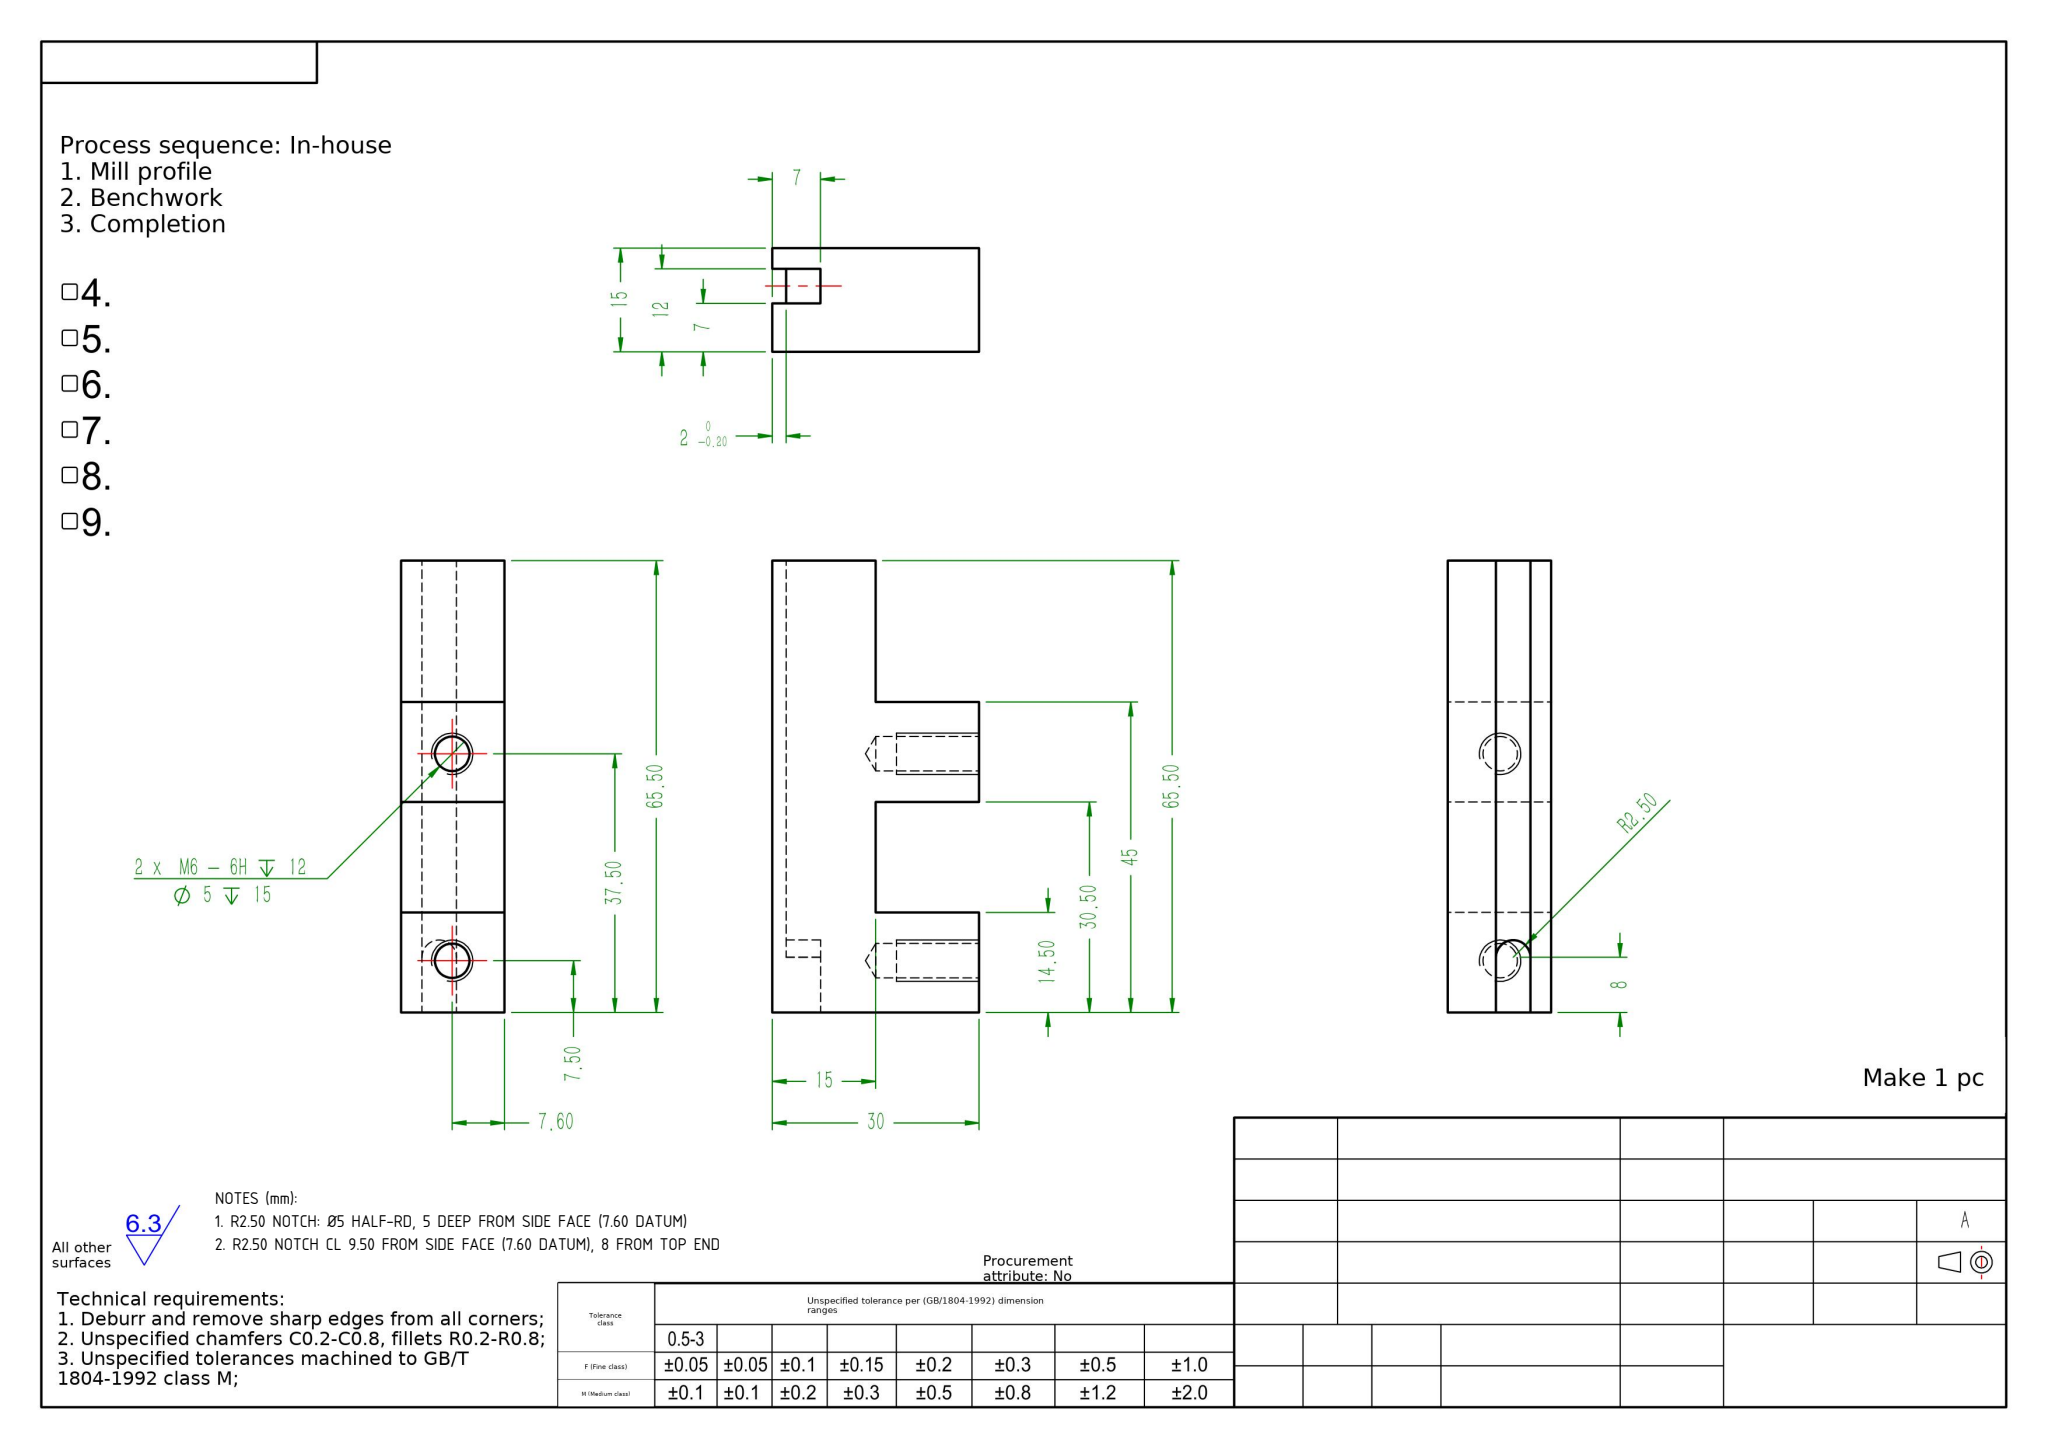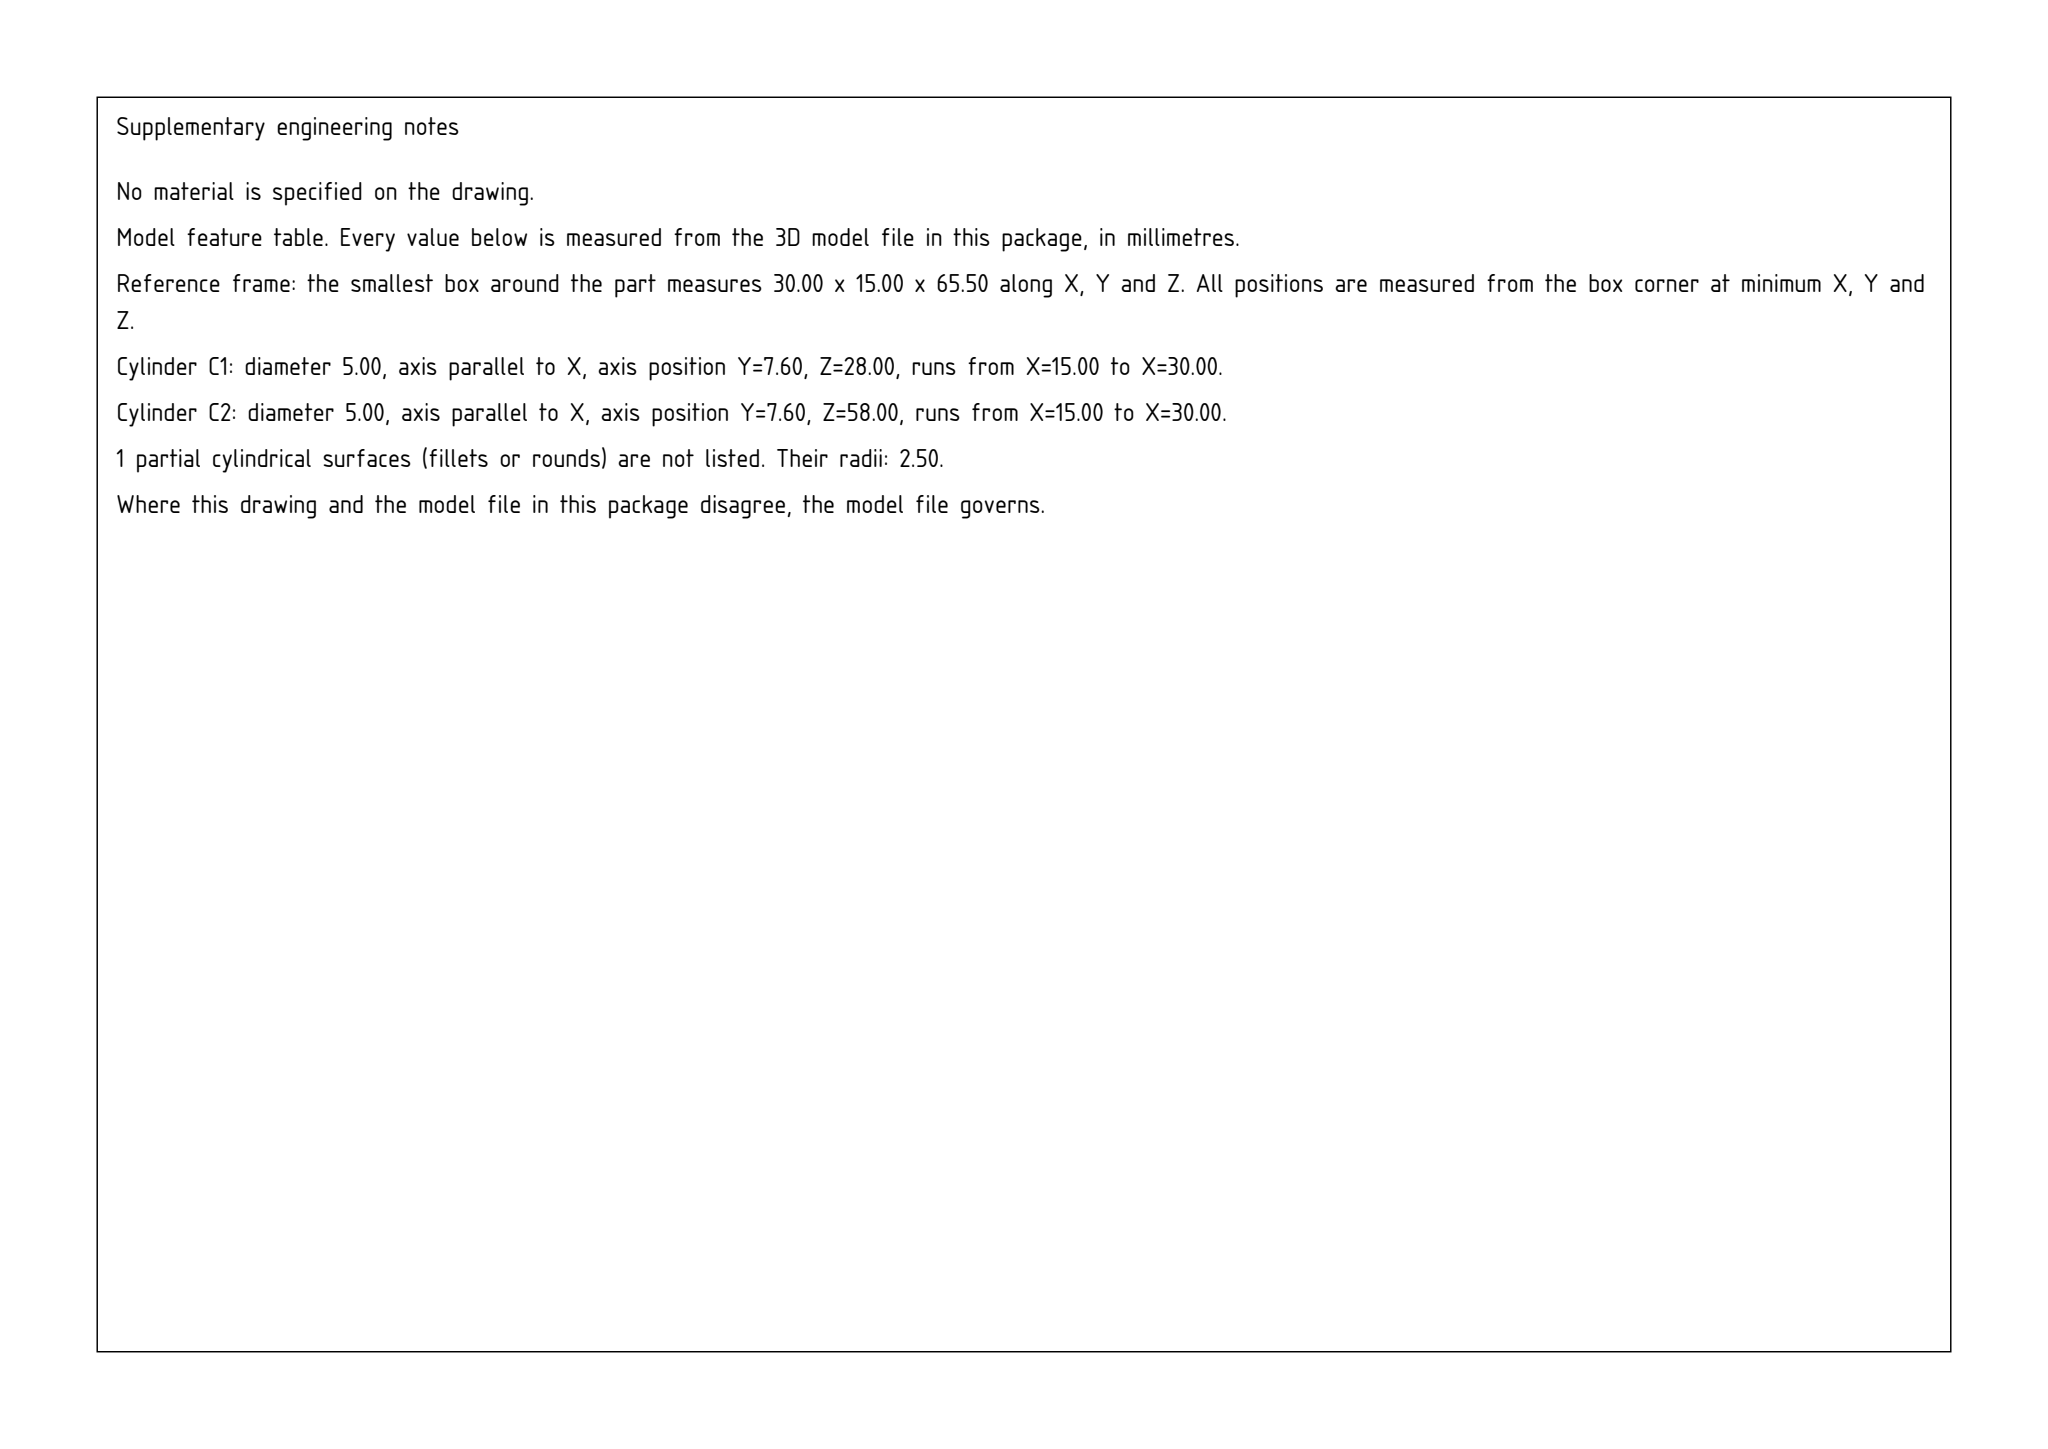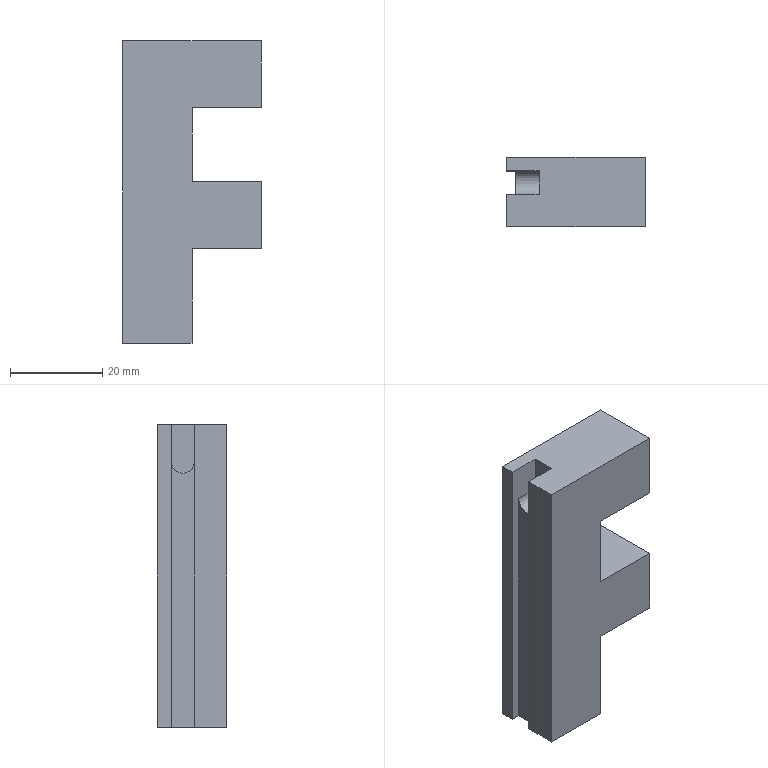Part | SolidWorks | mm | 1 solid | 26 faces | box 30 x 15 x 65.5 mm | volume 19750 mm3 | plane 17 | cylinder 5 | cone 4 | commonest cylinder face diameters 5 x5
Drawing notes:
R2.50 NOTCH: Ø5 HALF-RD, 5 DEEP FROM SIDE FACE (7.60 DATUM) | from the solid: cylinder dia 5.0, axis x, length 5.0 starting at x=0 face
R2.50 NOTCH CL 9.50 FROM SIDE FACE (7.60 DATUM), 8 FROM TOP END | from the solid: cylinder [5.0,'x',[null,9.5,57.5],5.0]; 65.5-57.5=8
build123d program:
from build123d import *

# Parameters (mm, degrees)
BOSS_EXTRUDE1_DEPTH   = 15
M6_TAPPED_HOLE1_D     = 5
M6_TAPPED_HOLE1_DEPTH = 15
M6_TAPPED_HOLE1_TIP   = 1.502
SKETCH4_W             = 65.5
SKETCH4_H             = 5
CUT_EXTRUDE1_DEPTH    = 2
CUT_EXTRUDE2_DEPTH    = 5


with BuildPart() as part:
    # Sketch1 → Boss-Extrude1 (new body)
    with BuildSketch(Plane(origin=(0, 0, 0), x_dir=(1, 0, 0), z_dir=(0, 1, 0))):
        Polygon((0, 0), (0, 65.5), (15, 65.5), (15, 45), (30, 45), (30, 30.5), (15, 30.5), (15, 14.5), (30, 14.5), (30, 0), align=None)
    extrude(amount=BOSS_EXTRUDE1_DEPTH)

    # M6 Tapped Hole1
    with Locations(Plane(origin=(30, 0, 0), x_dir=(0, 0, -1), z_dir=(1, 0, 0))):
        with Locations((7.5, 7.6), (37.5, 7.6)):
            Hole(M6_TAPPED_HOLE1_D / 2, depth=M6_TAPPED_HOLE1_DEPTH)
            with Locations((0, 0, -(M6_TAPPED_HOLE1_DEPTH + M6_TAPPED_HOLE1_TIP / 2))):  # 118° drill point
                Cone(0, M6_TAPPED_HOLE1_D / 2, M6_TAPPED_HOLE1_TIP, mode=Mode.SUBTRACT)

    # Sketch4 → Cut-Extrude1 (cut)
    with BuildSketch(Plane.ZY):
        with Locations((-32.75, 9.5)):
            Rectangle(SKETCH4_W, SKETCH4_H)
    extrude(amount=-CUT_EXTRUDE1_DEPTH, mode=Mode.SUBTRACT)

    # Sketch5 → Cut-Extrude2 (cut)
    with BuildSketch(Plane.ZY.offset(-2)):
        with BuildLine():
            Line((0, 7), (-8, 7))
            ThreePointArc((-8, 7), (-10.5, 9.5), (-8, 12))
            Line((-8, 12), (0, 12))
            ThreePointArc((0, 12), (2.5, 9.5), (0, 7))
        make_face()
    extrude(amount=-CUT_EXTRUDE2_DEPTH, mode=Mode.SUBTRACT)


solid = part.part
STEP:
#1=CARTESIAN_POINT('',(15.,7.6,-5.));
#2=VERTEX_POINT('',#1);
#3=CARTESIAN_POINT('',(15.,7.6,-10.));
#4=VERTEX_POINT('',#3);
#5=CARTESIAN_POINT('',(15.,7.6,-7.5));
#6=DIRECTION('',(1.,0.,-0.));
#7=DIRECTION('',(0.,0.,-1.));
#8=AXIS2_PLACEMENT_3D('',#5,#6,#7);
#9=CIRCLE('',#8,2.5);
#10=EDGE_CURVE('',#2,#4,#9,.T.);
#11=ORIENTED_EDGE('',*,*,#10,.F.);
#12=CARTESIAN_POINT('',(30.,7.6,-5.));
#13=VERTEX_POINT('',#12);
#14=CARTESIAN_POINT('',(30.,7.6,-5.));
#15=DIRECTION('',(1.,0.,-0.));
#16=VECTOR('',#15,1000.);
#17=LINE('',#14,#16);
#18=EDGE_CURVE('',#2,#13,#17,.T.);
#19=ORIENTED_EDGE('',*,*,#18,.T.);
#20=CARTESIAN_POINT('',(30.,7.6,-10.));
#21=VERTEX_POINT('',#20);
#22=CARTESIAN_POINT('',(30.,7.6,-7.5));
#23=DIRECTION('',(1.,0.,-0.));
#24=DIRECTION('',(0.,0.,-1.));
#25=AXIS2_PLACEMENT_3D('',#22,#23,#24);
#26=CIRCLE('',#25,2.5);
#27=EDGE_CURVE('',#13,#21,#26,.T.);
#28=ORIENTED_EDGE('',*,*,#27,.T.);
#29=CARTESIAN_POINT('',(30.,7.6,-10.));
#30=DIRECTION('',(1.,0.,-0.));
#31=VECTOR('',#30,1000.);
#32=LINE('',#29,#31);
#33=EDGE_CURVE('',#4,#21,#32,.T.);
#34=ORIENTED_EDGE('',*,*,#33,.F.);
#35=EDGE_LOOP('',(#11,#19,#28,#34));
#36=FACE_OUTER_BOUND('',#35,.T.);
#37=CARTESIAN_POINT('',(30.,7.6,-7.5));
#38=DIRECTION('',(1.,0.,-0.));
#39=DIRECTION('',(0.,0.,-1.));
#40=AXIS2_PLACEMENT_3D('',#37,#38,#39);
#41=CYLINDRICAL_SURFACE('',#40,2.5);
#42=ADVANCED_FACE('',(#36),#41,.F.);
#43=CARTESIAN_POINT('',(13.498,7.6,-7.5));
#44=VERTEX_POINT('',#43);
#45=CARTESIAN_POINT('',(15.,7.6,-10.));
#46=DIRECTION('',(0.515,0.,-0.8572));
#47=VECTOR('',#46,1000.);
#48=LINE('',#45,#47);
#49=EDGE_CURVE('',#44,#4,#48,.T.);
#50=ORIENTED_EDGE('',*,*,#49,.F.);
#51=CARTESIAN_POINT('',(15.,7.6,-5.));
#52=DIRECTION('',(0.515,0.,0.8572));
#53=VECTOR('',#52,1000.);
#54=LINE('',#51,#53);
#55=EDGE_CURVE('',#44,#2,#54,.T.);
#56=ORIENTED_EDGE('',*,*,#55,.T.);
#57=ORIENTED_EDGE('',*,*,#10,.T.);
#58=EDGE_LOOP('',(#50,#56,#57));
#59=FACE_OUTER_BOUND('',#58,.T.);
#60=CARTESIAN_POINT('',(15.,7.6,-7.5));
#61=DIRECTION('',(1.,0.,-0.));
#62=DIRECTION('',(0.,0.,-1.));
#63=AXIS2_PLACEMENT_3D('',#60,#61,#62);
#64=CONICAL_SURFACE('',#63,2.5,1.03);
#65=ADVANCED_FACE('',(#59),#64,.F.);
#66=CARTESIAN_POINT('',(15.,7.6,-35.));
#67=VERTEX_POINT('',#66);
#68=CARTESIAN_POINT('',(15.,7.6,-40.));
#69=VERTEX_POINT('',#68);
#70=CARTESIAN_POINT('',(15.,7.6,-37.5));
#71=DIRECTION('',(1.,0.,-0.));
#72=DIRECTION('',(0.,0.,-1.));
#73=AXIS2_PLACEMENT_3D('',#70,#71,#72);
#74=CIRCLE('',#73,2.5);
#75=EDGE_CURVE('',#67,#69,#74,.T.);
#76=ORIENTED_EDGE('',*,*,#75,.F.);
#77=CARTESIAN_POINT('',(30.,7.6,-35.));
#78=VERTEX_POINT('',#77);
#79=CARTESIAN_POINT('',(30.,7.6,-35.));
#80=DIRECTION('',(1.,0.,-0.));
#81=VECTOR('',#80,1000.);
#82=LINE('',#79,#81);
#83=EDGE_CURVE('',#67,#78,#82,.T.);
#84=ORIENTED_EDGE('',*,*,#83,.T.);
#85=CARTESIAN_POINT('',(30.,7.6,-40.));
#86=VERTEX_POINT('',#85);
#87=CARTESIAN_POINT('',(30.,7.6,-37.5));
#88=DIRECTION('',(1.,0.,-0.));
#89=DIRECTION('',(0.,0.,-1.));
#90=AXIS2_PLACEMENT_3D('',#87,#88,#89);
#91=CIRCLE('',#90,2.5);
#92=EDGE_CURVE('',#78,#86,#91,.T.);
#93=ORIENTED_EDGE('',*,*,#92,.T.);
#94=CARTESIAN_POINT('',(30.,7.6,-40.));
#95=DIRECTION('',(1.,0.,-0.));
#96=VECTOR('',#95,1000.);
#97=LINE('',#94,#96);
#98=EDGE_CURVE('',#69,#86,#97,.T.);
#99=ORIENTED_EDGE('',*,*,#98,.F.);
#100=EDGE_LOOP('',(#76,#84,#93,#99));
#101=FACE_OUTER_BOUND('',#100,.T.);
#102=CARTESIAN_POINT('',(30.,7.6,-37.5));
#103=DIRECTION('',(1.,0.,-0.));
#104=DIRECTION('',(0.,0.,-1.));
#105=AXIS2_PLACEMENT_3D('',#102,#103,#104);
#106=CYLINDRICAL_SURFACE('',#105,2.5);
#107=ADVANCED_FACE('',(#101),#106,.F.);
#108=CARTESIAN_POINT('',(13.498,7.6,-37.5));
#109=VERTEX_POINT('',#108);
#110=CARTESIAN_POINT('',(15.,7.6,-40.));
#111=DIRECTION('',(0.515,0.,-0.8572));
#112=VECTOR('',#111,1000.);
#113=LINE('',#110,#112);
#114=EDGE_CURVE('',#109,#69,#113,.T.);
#115=ORIENTED_EDGE('',*,*,#114,.F.);
#116=CARTESIAN_POINT('',(15.,7.6,-35.));
#117=DIRECTION('',(0.515,0.,0.8572));
#118=VECTOR('',#117,1000.);
#119=LINE('',#116,#118);
#120=EDGE_CURVE('',#109,#67,#119,.T.);
#121=ORIENTED_EDGE('',*,*,#120,.T.);
#122=ORIENTED_EDGE('',*,*,#75,.T.);
#123=EDGE_LOOP('',(#115,#121,#122));
#124=FACE_OUTER_BOUND('',#123,.T.);
#125=CARTESIAN_POINT('',(15.,7.6,-37.5));
#126=DIRECTION('',(1.,0.,-0.));
#127=DIRECTION('',(0.,0.,-1.));
#128=AXIS2_PLACEMENT_3D('',#125,#126,#127);
#129=CONICAL_SURFACE('',#128,2.5,1.03);
#130=ADVANCED_FACE('',(#124),#129,.F.);
#131=CARTESIAN_POINT('',(0.,15.,-65.5));
#132=VERTEX_POINT('',#131);
#133=CARTESIAN_POINT('',(0.,12.,-65.5));
#134=VERTEX_POINT('',#133);
#135=CARTESIAN_POINT('',(0.,15.,-65.5));
#136=DIRECTION('',(0.,-1.,0.));
#137=VECTOR('',#136,1000.);
#138=LINE('',#135,#137);
#139=EDGE_CURVE('',#132,#134,#138,.T.);
#140=ORIENTED_EDGE('',*,*,#139,.T.);
#141=CARTESIAN_POINT('',(0.,12.,0.));
#142=VERTEX_POINT('',#141);
#143=CARTESIAN_POINT('',(0.,12.,-65.5));
#144=DIRECTION('',(0.,0.,-1.));
#145=VECTOR('',#144,1000.);
#146=LINE('',#143,#145);
#147=EDGE_CURVE('',#142,#134,#146,.T.);
#148=ORIENTED_EDGE('',*,*,#147,.F.);
#149=CARTESIAN_POINT('',(0.,15.,0.));
#150=VERTEX_POINT('',#149);
#151=CARTESIAN_POINT('',(0.,15.,0.));
#152=DIRECTION('',(0.,-1.,0.));
#153=VECTOR('',#152,1000.);
#154=LINE('',#151,#153);
#155=EDGE_CURVE('',#150,#142,#154,.T.);
#156=ORIENTED_EDGE('',*,*,#155,.F.);
#157=CARTESIAN_POINT('',(0.,15.,0.));
#158=DIRECTION('',(0.,0.,1.));
#159=VECTOR('',#158,1000.);
#160=LINE('',#157,#159);
#161=EDGE_CURVE('',#132,#150,#160,.T.);
#162=ORIENTED_EDGE('',*,*,#161,.F.);
#163=EDGE_LOOP('',(#140,#148,#156,#162));
#164=FACE_OUTER_BOUND('',#163,.T.);
#165=CARTESIAN_POINT('',(0.,15.,0.));
#166=DIRECTION('',(1.,0.,0.));
#167=DIRECTION('',(0.,0.,-1.));
#168=AXIS2_PLACEMENT_3D('',#165,#166,#167);
#169=PLANE('',#168);
#170=ADVANCED_FACE('',(#164),#169,.F.);
#171=CARTESIAN_POINT('',(7.,7.,0.));
#172=VERTEX_POINT('',#171);
#173=CARTESIAN_POINT('',(7.,12.,0.));
#174=VERTEX_POINT('',#173);
#175=CARTESIAN_POINT('',(7.,15.,0.));
#176=DIRECTION('',(0.,1.,0.));
#177=VECTOR('',#176,1000.);
#178=LINE('',#175,#177);
#179=EDGE_CURVE('',#172,#174,#178,.T.);
#180=ORIENTED_EDGE('',*,*,#179,.F.);
#181=CARTESIAN_POINT('',(0.,7.,0.));
#182=VERTEX_POINT('',#181);
#183=CARTESIAN_POINT('',(2.,7.,0.));
#184=DIRECTION('',(-1.,0.,0.));
#185=VECTOR('',#184,1000.);
#186=LINE('',#183,#185);
#187=EDGE_CURVE('',#172,#182,#186,.T.);
#188=ORIENTED_EDGE('',*,*,#187,.T.);
#189=CARTESIAN_POINT('',(0.,0.,0.));
#190=VERTEX_POINT('',#189);
#191=CARTESIAN_POINT('',(0.,15.,0.));
#192=DIRECTION('',(0.,-1.,0.));
#193=VECTOR('',#192,1000.);
#194=LINE('',#191,#193);
#195=EDGE_CURVE('',#182,#190,#194,.T.);
#196=ORIENTED_EDGE('',*,*,#195,.T.);
#197=CARTESIAN_POINT('',(30.,0.,0.));
#198=VERTEX_POINT('',#197);
#199=CARTESIAN_POINT('',(30.,0.,0.));
#200=DIRECTION('',(1.,0.,0.));
#201=VECTOR('',#200,1000.);
#202=LINE('',#199,#201);
#203=EDGE_CURVE('',#190,#198,#202,.T.);
#204=ORIENTED_EDGE('',*,*,#203,.T.);
#205=CARTESIAN_POINT('',(30.,15.,0.));
#206=VERTEX_POINT('',#205);
#207=CARTESIAN_POINT('',(30.,15.,0.));
#208=DIRECTION('',(0.,-1.,0.));
#209=VECTOR('',#208,1000.);
#210=LINE('',#207,#209);
#211=EDGE_CURVE('',#206,#198,#210,.T.);
#212=ORIENTED_EDGE('',*,*,#211,.F.);
#213=CARTESIAN_POINT('',(30.,15.,0.));
#214=DIRECTION('',(1.,0.,0.));
#215=VECTOR('',#214,1000.);
#216=LINE('',#213,#215);
#217=EDGE_CURVE('',#150,#206,#216,.T.);
#218=ORIENTED_EDGE('',*,*,#217,.F.);
#219=ORIENTED_EDGE('',*,*,#155,.T.);
#220=CARTESIAN_POINT('',(2.,12.,0.));
#221=DIRECTION('',(-1.,0.,0.));
#222=VECTOR('',#221,1000.);
#223=LINE('',#220,#222);
#224=EDGE_CURVE('',#174,#142,#223,.T.);
#225=ORIENTED_EDGE('',*,*,#224,.F.);
#226=EDGE_LOOP('',(#180,#188,#196,#204,#212,#218,#219,#225));
#227=FACE_OUTER_BOUND('',#226,.T.);
#228=CARTESIAN_POINT('',(30.,15.,0.));
#229=DIRECTION('',(0.,0.,-1.));
#230=DIRECTION('',(-1.,0.,-0.));
#231=AXIS2_PLACEMENT_3D('',#228,#229,#230);
#232=PLANE('',#231);
#233=ADVANCED_FACE('',(#227),#232,.F.);
#234=CARTESIAN_POINT('',(30.,7.6,-7.5));
#235=DIRECTION('',(1.,0.,-0.));
#236=DIRECTION('',(0.,0.,-1.));
#237=AXIS2_PLACEMENT_3D('',#234,#235,#236);
#238=CIRCLE('',#237,2.5);
#239=EDGE_CURVE('',#21,#13,#238,.T.);
#240=ORIENTED_EDGE('',*,*,#239,.F.);
#241=ORIENTED_EDGE('',*,*,#27,.F.);
#242=EDGE_LOOP('',(#240,#241));
#243=FACE_BOUND('',#242,.T.);
#244=CARTESIAN_POINT('',(30.,0.,-14.5));
#245=VERTEX_POINT('',#244);
#246=CARTESIAN_POINT('',(30.,0.,-14.5));
#247=DIRECTION('',(-0.,0.,-1.));
#248=VECTOR('',#247,1000.);
#249=LINE('',#246,#248);
#250=EDGE_CURVE('',#198,#245,#249,.T.);
#251=ORIENTED_EDGE('',*,*,#250,.T.);
#252=CARTESIAN_POINT('',(30.,15.,-14.5));
#253=VERTEX_POINT('',#252);
#254=CARTESIAN_POINT('',(30.,15.,-14.5));
#255=DIRECTION('',(0.,-1.,0.));
#256=VECTOR('',#255,1000.);
#257=LINE('',#254,#256);
#258=EDGE_CURVE('',#253,#245,#257,.T.);
#259=ORIENTED_EDGE('',*,*,#258,.F.);
#260=CARTESIAN_POINT('',(30.,15.,-14.5));
#261=DIRECTION('',(-0.,0.,-1.));
#262=VECTOR('',#261,1000.);
#263=LINE('',#260,#262);
#264=EDGE_CURVE('',#206,#253,#263,.T.);
#265=ORIENTED_EDGE('',*,*,#264,.F.);
#266=ORIENTED_EDGE('',*,*,#211,.T.);
#267=EDGE_LOOP('',(#251,#259,#265,#266));
#268=FACE_OUTER_BOUND('',#267,.T.);
#269=CARTESIAN_POINT('',(30.,15.,-14.5));
#270=DIRECTION('',(-1.,0.,0.));
#271=DIRECTION('',(0.,0.,1.));
#272=AXIS2_PLACEMENT_3D('',#269,#270,#271);
#273=PLANE('',#272);
#274=ADVANCED_FACE('',(#243,#268),#273,.F.);
#275=CARTESIAN_POINT('',(15.,0.,-14.5));
#276=VERTEX_POINT('',#275);
#277=CARTESIAN_POINT('',(15.,0.,-14.5));
#278=DIRECTION('',(-1.,0.,0.));
#279=VECTOR('',#278,1000.);
#280=LINE('',#277,#279);
#281=EDGE_CURVE('',#245,#276,#280,.T.);
#282=ORIENTED_EDGE('',*,*,#281,.T.);
#283=CARTESIAN_POINT('',(15.,15.,-14.5));
#284=VERTEX_POINT('',#283);
#285=CARTESIAN_POINT('',(15.,15.,-14.5));
#286=DIRECTION('',(0.,-1.,0.));
#287=VECTOR('',#286,1000.);
#288=LINE('',#285,#287);
#289=EDGE_CURVE('',#284,#276,#288,.T.);
#290=ORIENTED_EDGE('',*,*,#289,.F.);
#291=CARTESIAN_POINT('',(15.,15.,-14.5));
#292=DIRECTION('',(-1.,0.,0.));
#293=VECTOR('',#292,1000.);
#294=LINE('',#291,#293);
#295=EDGE_CURVE('',#253,#284,#294,.T.);
#296=ORIENTED_EDGE('',*,*,#295,.F.);
#297=ORIENTED_EDGE('',*,*,#258,.T.);
#298=EDGE_LOOP('',(#282,#290,#296,#297));
#299=FACE_OUTER_BOUND('',#298,.T.);
#300=CARTESIAN_POINT('',(15.,15.,-14.5));
#301=DIRECTION('',(0.,0.,1.));
#302=DIRECTION('',(1.,0.,0.));
#303=AXIS2_PLACEMENT_3D('',#300,#301,#302);
#304=PLANE('',#303);
#305=ADVANCED_FACE('',(#299),#304,.F.);
#306=CARTESIAN_POINT('',(15.,0.,-30.5));
#307=VERTEX_POINT('',#306);
#308=CARTESIAN_POINT('',(15.,0.,-30.5));
#309=DIRECTION('',(-0.,0.,-1.));
#310=VECTOR('',#309,1000.);
#311=LINE('',#308,#310);
#312=EDGE_CURVE('',#276,#307,#311,.T.);
#313=ORIENTED_EDGE('',*,*,#312,.T.);
#314=CARTESIAN_POINT('',(15.,15.,-30.5));
#315=VERTEX_POINT('',#314);
#316=CARTESIAN_POINT('',(15.,15.,-30.5));
#317=DIRECTION('',(0.,-1.,0.));
#318=VECTOR('',#317,1000.);
#319=LINE('',#316,#318);
#320=EDGE_CURVE('',#315,#307,#319,.T.);
#321=ORIENTED_EDGE('',*,*,#320,.F.);
#322=CARTESIAN_POINT('',(15.,15.,-30.5));
#323=DIRECTION('',(-0.,0.,-1.));
#324=VECTOR('',#323,1000.);
#325=LINE('',#322,#324);
#326=EDGE_CURVE('',#284,#315,#325,.T.);
#327=ORIENTED_EDGE('',*,*,#326,.F.);
#328=ORIENTED_EDGE('',*,*,#289,.T.);
#329=EDGE_LOOP('',(#313,#321,#327,#328));
#330=FACE_OUTER_BOUND('',#329,.T.);
#331=CARTESIAN_POINT('',(15.,15.,-30.5));
#332=DIRECTION('',(-1.,0.,0.));
#333=DIRECTION('',(0.,0.,1.));
#334=AXIS2_PLACEMENT_3D('',#331,#332,#333);
#335=PLANE('',#334);
#336=ADVANCED_FACE('',(#330),#335,.F.);
#337=CARTESIAN_POINT('',(30.,0.,-30.5));
#338=VERTEX_POINT('',#337);
#339=CARTESIAN_POINT('',(30.,0.,-30.5));
#340=DIRECTION('',(1.,0.,-0.));
#341=VECTOR('',#340,1000.);
#342=LINE('',#339,#341);
#343=EDGE_CURVE('',#307,#338,#342,.T.);
#344=ORIENTED_EDGE('',*,*,#343,.T.);
#345=CARTESIAN_POINT('',(30.,15.,-30.5));
#346=VERTEX_POINT('',#345);
#347=CARTESIAN_POINT('',(30.,15.,-30.5));
#348=DIRECTION('',(0.,-1.,0.));
#349=VECTOR('',#348,1000.);
#350=LINE('',#347,#349);
#351=EDGE_CURVE('',#346,#338,#350,.T.);
#352=ORIENTED_EDGE('',*,*,#351,.F.);
#353=CARTESIAN_POINT('',(30.,15.,-30.5));
#354=DIRECTION('',(1.,0.,-0.));
#355=VECTOR('',#354,1000.);
#356=LINE('',#353,#355);
#357=EDGE_CURVE('',#315,#346,#356,.T.);
#358=ORIENTED_EDGE('',*,*,#357,.F.);
#359=ORIENTED_EDGE('',*,*,#320,.T.);
#360=EDGE_LOOP('',(#344,#352,#358,#359));
#361=FACE_OUTER_BOUND('',#360,.T.);
#362=CARTESIAN_POINT('',(30.,15.,-30.5));
#363=DIRECTION('',(-0.,0.,-1.));
#364=DIRECTION('',(-1.,0.,0.));
#365=AXIS2_PLACEMENT_3D('',#362,#363,#364);
#366=PLANE('',#365);
#367=ADVANCED_FACE('',(#361),#366,.F.);
#368=CARTESIAN_POINT('',(30.,7.6,-37.5));
#369=DIRECTION('',(1.,0.,-0.));
#370=DIRECTION('',(0.,0.,-1.));
#371=AXIS2_PLACEMENT_3D('',#368,#369,#370);
#372=CIRCLE('',#371,2.5);
#373=EDGE_CURVE('',#86,#78,#372,.T.);
#374=ORIENTED_EDGE('',*,*,#373,.F.);
#375=ORIENTED_EDGE('',*,*,#92,.F.);
#376=EDGE_LOOP('',(#374,#375));
#377=FACE_BOUND('',#376,.T.);
#378=CARTESIAN_POINT('',(30.,0.,-45.));
#379=VERTEX_POINT('',#378);
#380=CARTESIAN_POINT('',(30.,0.,-45.));
#381=DIRECTION('',(-0.,0.,-1.));
#382=VECTOR('',#381,1000.);
#383=LINE('',#380,#382);
#384=EDGE_CURVE('',#338,#379,#383,.T.);
#385=ORIENTED_EDGE('',*,*,#384,.T.);
#386=CARTESIAN_POINT('',(30.,15.,-45.));
#387=VERTEX_POINT('',#386);
#388=CARTESIAN_POINT('',(30.,15.,-45.));
#389=DIRECTION('',(0.,-1.,0.));
#390=VECTOR('',#389,1000.);
#391=LINE('',#388,#390);
#392=EDGE_CURVE('',#387,#379,#391,.T.);
#393=ORIENTED_EDGE('',*,*,#392,.F.);
#394=CARTESIAN_POINT('',(30.,15.,-45.));
#395=DIRECTION('',(-0.,0.,-1.));
#396=VECTOR('',#395,1000.);
#397=LINE('',#394,#396);
#398=EDGE_CURVE('',#346,#387,#397,.T.);
#399=ORIENTED_EDGE('',*,*,#398,.F.);
#400=ORIENTED_EDGE('',*,*,#351,.T.);
#401=EDGE_LOOP('',(#385,#393,#399,#400));
#402=FACE_OUTER_BOUND('',#401,.T.);
#403=CARTESIAN_POINT('',(30.,15.,-45.));
#404=DIRECTION('',(-1.,0.,0.));
#405=DIRECTION('',(0.,0.,1.));
#406=AXIS2_PLACEMENT_3D('',#403,#404,#405);
#407=PLANE('',#406);
#408=ADVANCED_FACE('',(#377,#402),#407,.F.);
#409=CARTESIAN_POINT('',(15.,0.,-45.));
#410=VERTEX_POINT('',#409);
#411=CARTESIAN_POINT('',(15.,0.,-45.));
#412=DIRECTION('',(-1.,0.,0.));
#413=VECTOR('',#412,1000.);
#414=LINE('',#411,#413);
#415=EDGE_CURVE('',#379,#410,#414,.T.);
#416=ORIENTED_EDGE('',*,*,#415,.T.);
#417=CARTESIAN_POINT('',(15.,15.,-45.));
#418=VERTEX_POINT('',#417);
#419=CARTESIAN_POINT('',(15.,15.,-45.));
#420=DIRECTION('',(0.,-1.,0.));
#421=VECTOR('',#420,1000.);
#422=LINE('',#419,#421);
#423=EDGE_CURVE('',#418,#410,#422,.T.);
#424=ORIENTED_EDGE('',*,*,#423,.F.);
#425=CARTESIAN_POINT('',(15.,15.,-45.));
#426=DIRECTION('',(-1.,0.,0.));
#427=VECTOR('',#426,1000.);
#428=LINE('',#425,#427);
#429=EDGE_CURVE('',#387,#418,#428,.T.);
#430=ORIENTED_EDGE('',*,*,#429,.F.);
#431=ORIENTED_EDGE('',*,*,#392,.T.);
#432=EDGE_LOOP('',(#416,#424,#430,#431));
#433=FACE_OUTER_BOUND('',#432,.T.);
#434=CARTESIAN_POINT('',(15.,15.,-45.));
#435=DIRECTION('',(0.,0.,1.));
#436=DIRECTION('',(1.,0.,0.));
#437=AXIS2_PLACEMENT_3D('',#434,#435,#436);
#438=PLANE('',#437);
#439=ADVANCED_FACE('',(#433),#438,.F.);
#440=CARTESIAN_POINT('',(15.,0.,-65.5));
#441=VERTEX_POINT('',#440);
#442=CARTESIAN_POINT('',(15.,0.,-65.5));
#443=DIRECTION('',(-0.,0.,-1.));
#444=VECTOR('',#443,1000.);
#445=LINE('',#442,#444);
#446=EDGE_CURVE('',#410,#441,#445,.T.);
#447=ORIENTED_EDGE('',*,*,#446,.T.);
#448=CARTESIAN_POINT('',(15.,15.,-65.5));
#449=VERTEX_POINT('',#448);
#450=CARTESIAN_POINT('',(15.,15.,-65.5));
#451=DIRECTION('',(0.,-1.,0.));
#452=VECTOR('',#451,1000.);
#453=LINE('',#450,#452);
#454=EDGE_CURVE('',#449,#441,#453,.T.);
#455=ORIENTED_EDGE('',*,*,#454,.F.);
#456=CARTESIAN_POINT('',(15.,15.,-65.5));
#457=DIRECTION('',(-0.,0.,-1.));
#458=VECTOR('',#457,1000.);
#459=LINE('',#456,#458);
#460=EDGE_CURVE('',#418,#449,#459,.T.);
#461=ORIENTED_EDGE('',*,*,#460,.F.);
#462=ORIENTED_EDGE('',*,*,#423,.T.);
#463=EDGE_LOOP('',(#447,#455,#461,#462));
#464=FACE_OUTER_BOUND('',#463,.T.);
#465=CARTESIAN_POINT('',(15.,15.,-65.5));
#466=DIRECTION('',(-1.,0.,0.));
#467=DIRECTION('',(0.,0.,1.));
#468=AXIS2_PLACEMENT_3D('',#465,#466,#467);
#469=PLANE('',#468);
#470=ADVANCED_FACE('',(#464),#469,.F.);
#471=CARTESIAN_POINT('',(2.,12.,-65.5));
#472=VERTEX_POINT('',#471);
#473=CARTESIAN_POINT('',(2.,7.,-65.5));
#474=VERTEX_POINT('',#473);
#475=CARTESIAN_POINT('',(2.,12.,-65.5));
#476=DIRECTION('',(0.,-1.,0.));
#477=VECTOR('',#476,1000.);
#478=LINE('',#475,#477);
#479=EDGE_CURVE('',#472,#474,#478,.T.);
#480=ORIENTED_EDGE('',*,*,#479,.F.);
#481=CARTESIAN_POINT('',(2.,12.,-65.5));
#482=DIRECTION('',(-1.,0.,0.));
#483=VECTOR('',#482,1000.);
#484=LINE('',#481,#483);
#485=EDGE_CURVE('',#472,#134,#484,.T.);
#486=ORIENTED_EDGE('',*,*,#485,.T.);
#487=ORIENTED_EDGE('',*,*,#139,.F.);
#488=CARTESIAN_POINT('',(0.,15.,-65.5));
#489=DIRECTION('',(-1.,0.,0.));
#490=VECTOR('',#489,1000.);
#491=LINE('',#488,#490);
#492=EDGE_CURVE('',#449,#132,#491,.T.);
#493=ORIENTED_EDGE('',*,*,#492,.F.);
#494=ORIENTED_EDGE('',*,*,#454,.T.);
#495=CARTESIAN_POINT('',(0.,0.,-65.5));
#496=VERTEX_POINT('',#495);
#497=CARTESIAN_POINT('',(0.,0.,-65.5));
#498=DIRECTION('',(-1.,0.,0.));
#499=VECTOR('',#498,1000.);
#500=LINE('',#497,#499);
#501=EDGE_CURVE('',#441,#496,#500,.T.);
#502=ORIENTED_EDGE('',*,*,#501,.T.);
#503=CARTESIAN_POINT('',(0.,7.,-65.5));
#504=VERTEX_POINT('',#503);
#505=CARTESIAN_POINT('',(0.,15.,-65.5));
#506=DIRECTION('',(0.,-1.,0.));
#507=VECTOR('',#506,1000.);
#508=LINE('',#505,#507);
#509=EDGE_CURVE('',#504,#496,#508,.T.);
#510=ORIENTED_EDGE('',*,*,#509,.F.);
#511=CARTESIAN_POINT('',(2.,7.,-65.5));
#512=DIRECTION('',(-1.,0.,0.));
#513=VECTOR('',#512,1000.);
#514=LINE('',#511,#513);
#515=EDGE_CURVE('',#474,#504,#514,.T.);
#516=ORIENTED_EDGE('',*,*,#515,.F.);
#517=EDGE_LOOP('',(#480,#486,#487,#493,#494,#502,#510,#516));
#518=FACE_OUTER_BOUND('',#517,.T.);
#519=CARTESIAN_POINT('',(0.,15.,-65.5));
#520=DIRECTION('',(0.,0.,1.));
#521=DIRECTION('',(1.,0.,0.));
#522=AXIS2_PLACEMENT_3D('',#519,#520,#521);
#523=PLANE('',#522);
#524=ADVANCED_FACE('',(#518),#523,.F.);
#525=ORIENTED_EDGE('',*,*,#195,.F.);
#526=CARTESIAN_POINT('',(0.,7.,-65.5));
#527=DIRECTION('',(0.,0.,1.));
#528=VECTOR('',#527,1000.);
#529=LINE('',#526,#528);
#530=EDGE_CURVE('',#504,#182,#529,.T.);
#531=ORIENTED_EDGE('',*,*,#530,.F.);
#532=ORIENTED_EDGE('',*,*,#509,.T.);
#533=CARTESIAN_POINT('',(0.,0.,0.));
#534=DIRECTION('',(0.,0.,1.));
#535=VECTOR('',#534,1000.);
#536=LINE('',#533,#535);
#537=EDGE_CURVE('',#496,#190,#536,.T.);
#538=ORIENTED_EDGE('',*,*,#537,.T.);
#539=EDGE_LOOP('',(#525,#531,#532,#538));
#540=FACE_OUTER_BOUND('',#539,.T.);
#541=CARTESIAN_POINT('',(0.,15.,0.));
#542=DIRECTION('',(1.,0.,0.));
#543=DIRECTION('',(0.,0.,-1.));
#544=AXIS2_PLACEMENT_3D('',#541,#542,#543);
#545=PLANE('',#544);
#546=ADVANCED_FACE('',(#540),#545,.F.);
#547=ORIENTED_EDGE('',*,*,#217,.T.);
#548=ORIENTED_EDGE('',*,*,#264,.T.);
#549=ORIENTED_EDGE('',*,*,#295,.T.);
#550=ORIENTED_EDGE('',*,*,#326,.T.);
#551=ORIENTED_EDGE('',*,*,#357,.T.);
#552=ORIENTED_EDGE('',*,*,#398,.T.);
#553=ORIENTED_EDGE('',*,*,#429,.T.);
#554=ORIENTED_EDGE('',*,*,#460,.T.);
#555=ORIENTED_EDGE('',*,*,#492,.T.);
#556=ORIENTED_EDGE('',*,*,#161,.T.);
#557=EDGE_LOOP('',(#547,#548,#549,#550,#551,#552,#553,#554,#555,#556));
#558=FACE_OUTER_BOUND('',#557,.T.);
#559=CARTESIAN_POINT('',(0.,15.,0.));
#560=DIRECTION('',(0.,-1.,0.));
#561=DIRECTION('',(0.,0.,-1.));
#562=AXIS2_PLACEMENT_3D('',#559,#560,#561);
#563=PLANE('',#562);
#564=ADVANCED_FACE('',(#558),#563,.F.);
#565=ORIENTED_EDGE('',*,*,#203,.F.);
#566=ORIENTED_EDGE('',*,*,#537,.F.);
#567=ORIENTED_EDGE('',*,*,#501,.F.);
#568=ORIENTED_EDGE('',*,*,#446,.F.);
#569=ORIENTED_EDGE('',*,*,#415,.F.);
#570=ORIENTED_EDGE('',*,*,#384,.F.);
#571=ORIENTED_EDGE('',*,*,#343,.F.);
#572=ORIENTED_EDGE('',*,*,#312,.F.);
#573=ORIENTED_EDGE('',*,*,#281,.F.);
#574=ORIENTED_EDGE('',*,*,#250,.F.);
#575=EDGE_LOOP('',(#565,#566,#567,#568,#569,#570,#571,#572,#573,#574));
#576=FACE_OUTER_BOUND('',#575,.T.);
#577=CARTESIAN_POINT('',(0.,0.,0.));
#578=DIRECTION('',(0.,-1.,0.));
#579=DIRECTION('',(0.,0.,-1.));
#580=AXIS2_PLACEMENT_3D('',#577,#578,#579);
#581=PLANE('',#580);
#582=ADVANCED_FACE('',(#576),#581,.T.);
#583=ORIENTED_EDGE('',*,*,#120,.F.);
#584=ORIENTED_EDGE('',*,*,#114,.T.);
#585=CARTESIAN_POINT('',(15.,7.6,-37.5));
#586=DIRECTION('',(1.,0.,-0.));
#587=DIRECTION('',(0.,0.,-1.));
#588=AXIS2_PLACEMENT_3D('',#585,#586,#587);
#589=CIRCLE('',#588,2.5);
#590=EDGE_CURVE('',#69,#67,#589,.T.);
#591=ORIENTED_EDGE('',*,*,#590,.T.);
#592=EDGE_LOOP('',(#583,#584,#591));
#593=FACE_OUTER_BOUND('',#592,.T.);
#594=CARTESIAN_POINT('',(15.,7.6,-37.5));
#595=DIRECTION('',(1.,0.,-0.));
#596=DIRECTION('',(0.,0.,-1.));
#597=AXIS2_PLACEMENT_3D('',#594,#595,#596);
#598=CONICAL_SURFACE('',#597,2.5,1.03);
#599=ADVANCED_FACE('',(#593),#598,.F.);
#600=ORIENTED_EDGE('',*,*,#83,.F.);
#601=ORIENTED_EDGE('',*,*,#590,.F.);
#602=ORIENTED_EDGE('',*,*,#98,.T.);
#603=ORIENTED_EDGE('',*,*,#373,.T.);
#604=EDGE_LOOP('',(#600,#601,#602,#603));
#605=FACE_OUTER_BOUND('',#604,.T.);
#606=CARTESIAN_POINT('',(30.,7.6,-37.5));
#607=DIRECTION('',(1.,0.,-0.));
#608=DIRECTION('',(0.,0.,-1.));
#609=AXIS2_PLACEMENT_3D('',#606,#607,#608);
#610=CYLINDRICAL_SURFACE('',#609,2.5);
#611=ADVANCED_FACE('',(#605),#610,.F.);
#612=ORIENTED_EDGE('',*,*,#55,.F.);
#613=ORIENTED_EDGE('',*,*,#49,.T.);
#614=CARTESIAN_POINT('',(15.,7.6,-7.5));
#615=DIRECTION('',(1.,0.,-0.));
#616=DIRECTION('',(0.,0.,-1.));
#617=AXIS2_PLACEMENT_3D('',#614,#615,#616);
#618=CIRCLE('',#617,2.5);
#619=EDGE_CURVE('',#4,#2,#618,.T.);
#620=ORIENTED_EDGE('',*,*,#619,.T.);
#621=EDGE_LOOP('',(#612,#613,#620));
#622=FACE_OUTER_BOUND('',#621,.T.);
#623=CARTESIAN_POINT('',(15.,7.6,-7.5));
#624=DIRECTION('',(1.,0.,-0.));
#625=DIRECTION('',(0.,0.,-1.));
#626=AXIS2_PLACEMENT_3D('',#623,#624,#625);
#627=CONICAL_SURFACE('',#626,2.5,1.03);
#628=ADVANCED_FACE('',(#622),#627,.F.);
#629=ORIENTED_EDGE('',*,*,#18,.F.);
#630=ORIENTED_EDGE('',*,*,#619,.F.);
#631=ORIENTED_EDGE('',*,*,#33,.T.);
#632=ORIENTED_EDGE('',*,*,#239,.T.);
#633=EDGE_LOOP('',(#629,#630,#631,#632));
#634=FACE_OUTER_BOUND('',#633,.T.);
#635=CARTESIAN_POINT('',(30.,7.6,-7.5));
#636=DIRECTION('',(1.,0.,-0.));
#637=DIRECTION('',(0.,0.,-1.));
#638=AXIS2_PLACEMENT_3D('',#635,#636,#637);
#639=CYLINDRICAL_SURFACE('',#638,2.5);
#640=ADVANCED_FACE('',(#634),#639,.F.);
#641=ORIENTED_EDGE('',*,*,#147,.T.);
#642=ORIENTED_EDGE('',*,*,#485,.F.);
#643=CARTESIAN_POINT('',(2.,12.,-8.));
#644=VERTEX_POINT('',#643);
#645=CARTESIAN_POINT('',(2.,12.,-65.5));
#646=DIRECTION('',(0.,0.,-1.));
#647=VECTOR('',#646,1000.);
#648=LINE('',#645,#647);
#649=EDGE_CURVE('',#644,#472,#648,.T.);
#650=ORIENTED_EDGE('',*,*,#649,.F.);
#651=CARTESIAN_POINT('',(7.,12.,-8.));
#652=VERTEX_POINT('',#651);
#653=CARTESIAN_POINT('',(7.,12.,-8.));
#654=DIRECTION('',(-1.,0.,0.));
#655=VECTOR('',#654,1000.);
#656=LINE('',#653,#655);
#657=EDGE_CURVE('',#652,#644,#656,.T.);
#658=ORIENTED_EDGE('',*,*,#657,.F.);
#659=CARTESIAN_POINT('',(7.,12.,0.));
#660=DIRECTION('',(0.,0.,-1.));
#661=VECTOR('',#660,1000.);
#662=LINE('',#659,#661);
#663=EDGE_CURVE('',#174,#652,#662,.T.);
#664=ORIENTED_EDGE('',*,*,#663,.F.);
#665=ORIENTED_EDGE('',*,*,#224,.T.);
#666=EDGE_LOOP('',(#641,#642,#650,#658,#664,#665));
#667=FACE_OUTER_BOUND('',#666,.T.);
#668=CARTESIAN_POINT('',(2.,12.,-65.5));
#669=DIRECTION('',(0.,1.,0.));
#670=DIRECTION('',(0.,0.,1.));
#671=AXIS2_PLACEMENT_3D('',#668,#669,#670);
#672=PLANE('',#671);
#673=ADVANCED_FACE('',(#667),#672,.F.);
#674=ORIENTED_EDGE('',*,*,#530,.T.);
#675=ORIENTED_EDGE('',*,*,#187,.F.);
#676=CARTESIAN_POINT('',(7.,7.,-8.));
#677=VERTEX_POINT('',#676);
#678=CARTESIAN_POINT('',(7.,7.,0.));
#679=DIRECTION('',(0.,0.,1.));
#680=VECTOR('',#679,1000.);
#681=LINE('',#678,#680);
#682=EDGE_CURVE('',#677,#172,#681,.T.);
#683=ORIENTED_EDGE('',*,*,#682,.F.);
#684=CARTESIAN_POINT('',(2.,7.,-8.));
#685=VERTEX_POINT('',#684);
#686=CARTESIAN_POINT('',(7.,7.,-8.));
#687=DIRECTION('',(-1.,0.,0.));
#688=VECTOR('',#687,1000.);
#689=LINE('',#686,#688);
#690=EDGE_CURVE('',#677,#685,#689,.T.);
#691=ORIENTED_EDGE('',*,*,#690,.T.);
#692=CARTESIAN_POINT('',(2.,7.,-65.5));
#693=DIRECTION('',(0.,0.,1.));
#694=VECTOR('',#693,1000.);
#695=LINE('',#692,#694);
#696=EDGE_CURVE('',#474,#685,#695,.T.);
#697=ORIENTED_EDGE('',*,*,#696,.F.);
#698=ORIENTED_EDGE('',*,*,#515,.T.);
#699=EDGE_LOOP('',(#674,#675,#683,#691,#697,#698));
#700=FACE_OUTER_BOUND('',#699,.T.);
#701=CARTESIAN_POINT('',(2.,7.,-65.5));
#702=DIRECTION('',(0.,-1.,0.));
#703=DIRECTION('',(0.,0.,-1.));
#704=AXIS2_PLACEMENT_3D('',#701,#702,#703);
#705=PLANE('',#704);
#706=ADVANCED_FACE('',(#700),#705,.F.);
#707=CARTESIAN_POINT('',(2.,9.5,-8.));
#708=DIRECTION('',(-1.,0.,0.));
#709=DIRECTION('',(0.,0.,1.));
#710=AXIS2_PLACEMENT_3D('',#707,#708,#709);
#711=CIRCLE('',#710,2.5);
#712=EDGE_CURVE('',#644,#685,#711,.T.);
#713=ORIENTED_EDGE('',*,*,#712,.F.);
#714=ORIENTED_EDGE('',*,*,#649,.T.);
#715=ORIENTED_EDGE('',*,*,#479,.T.);
#716=ORIENTED_EDGE('',*,*,#696,.T.);
#717=EDGE_LOOP('',(#713,#714,#715,#716));
#718=FACE_OUTER_BOUND('',#717,.T.);
#719=CARTESIAN_POINT('',(2.,0.,0.));
#720=DIRECTION('',(-1.,0.,0.));
#721=DIRECTION('',(0.,0.,1.));
#722=AXIS2_PLACEMENT_3D('',#719,#720,#721);
#723=PLANE('',#722);
#724=ADVANCED_FACE('',(#718),#723,.T.);
#725=ORIENTED_EDGE('',*,*,#179,.T.);
#726=ORIENTED_EDGE('',*,*,#663,.T.);
#727=CARTESIAN_POINT('',(7.,9.5,-8.));
#728=DIRECTION('',(-1.,0.,0.));
#729=DIRECTION('',(0.,0.,1.));
#730=AXIS2_PLACEMENT_3D('',#727,#728,#729);
#731=CIRCLE('',#730,2.5);
#732=EDGE_CURVE('',#652,#677,#731,.T.);
#733=ORIENTED_EDGE('',*,*,#732,.T.);
#734=ORIENTED_EDGE('',*,*,#682,.T.);
#735=EDGE_LOOP('',(#725,#726,#733,#734));
#736=FACE_OUTER_BOUND('',#735,.T.);
#737=CARTESIAN_POINT('',(7.,9.5,0.));
#738=DIRECTION('',(-1.,0.,0.));
#739=DIRECTION('',(0.,0.,1.));
#740=AXIS2_PLACEMENT_3D('',#737,#738,#739);
#741=PLANE('',#740);
#742=ADVANCED_FACE('',(#736),#741,.T.);
#743=ORIENTED_EDGE('',*,*,#712,.T.);
#744=ORIENTED_EDGE('',*,*,#690,.F.);
#745=ORIENTED_EDGE('',*,*,#732,.F.);
#746=ORIENTED_EDGE('',*,*,#657,.T.);
#747=EDGE_LOOP('',(#743,#744,#745,#746));
#748=FACE_OUTER_BOUND('',#747,.T.);
#749=CARTESIAN_POINT('',(7.,9.5,-8.));
#750=DIRECTION('',(-1.,0.,0.));
#751=DIRECTION('',(0.,0.,1.));
#752=AXIS2_PLACEMENT_3D('',#749,#750,#751);
#753=CYLINDRICAL_SURFACE('',#752,2.5);
#754=ADVANCED_FACE('',(#748),#753,.F.);
#755=CLOSED_SHELL('',(#42,#65,#107,#130,#170,#233,#274,#305,#336,#367,#408,#439,#470,#524,#546,#564,#582,#599,#611,#628,#640,#673,#706,#724,#742,#754));
#756=MANIFOLD_SOLID_BREP('',#755);
#757=CARTESIAN_POINT('',(0.,0.,0.));
#758=DIRECTION('',(0.,0.,1.));
#759=DIRECTION('',(1.,0.,0.));
#760=AXIS2_PLACEMENT_3D('',#757,#758,#759);
#761=(LENGTH_UNIT()NAMED_UNIT(*)SI_UNIT(.MILLI.,.METRE.));
#762=UNCERTAINTY_MEASURE_WITH_UNIT(LENGTH_MEASURE(0.00001),#761,'','');
#763=(NAMED_UNIT(*)PLANE_ANGLE_UNIT()SI_UNIT($,.RADIAN.));
#764=(NAMED_UNIT(*)SI_UNIT($,.STERADIAN.)SOLID_ANGLE_UNIT());
#765=(GEOMETRIC_REPRESENTATION_CONTEXT(3)GLOBAL_UNCERTAINTY_ASSIGNED_CONTEXT((#762))GLOBAL_UNIT_ASSIGNED_CONTEXT((#761,#763,#764))REPRESENTATION_CONTEXT('',''));
#766=ADVANCED_BREP_SHAPE_REPRESENTATION('',(#756,#760),#765);